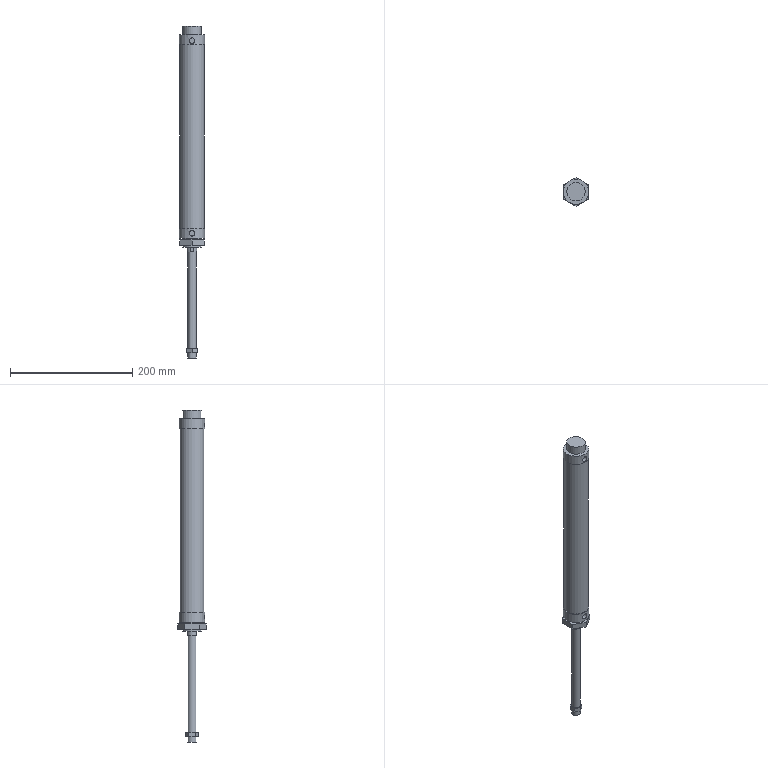Component | NX | COLUMN_CYL | 1 solid | 40 faces | volume 476516 mm3 | plane 28 | cylinder 12 | commonest cylinder face diameters 30 x3 41.6 x2 14 x2 16 x2 9.1 x2 40 x1